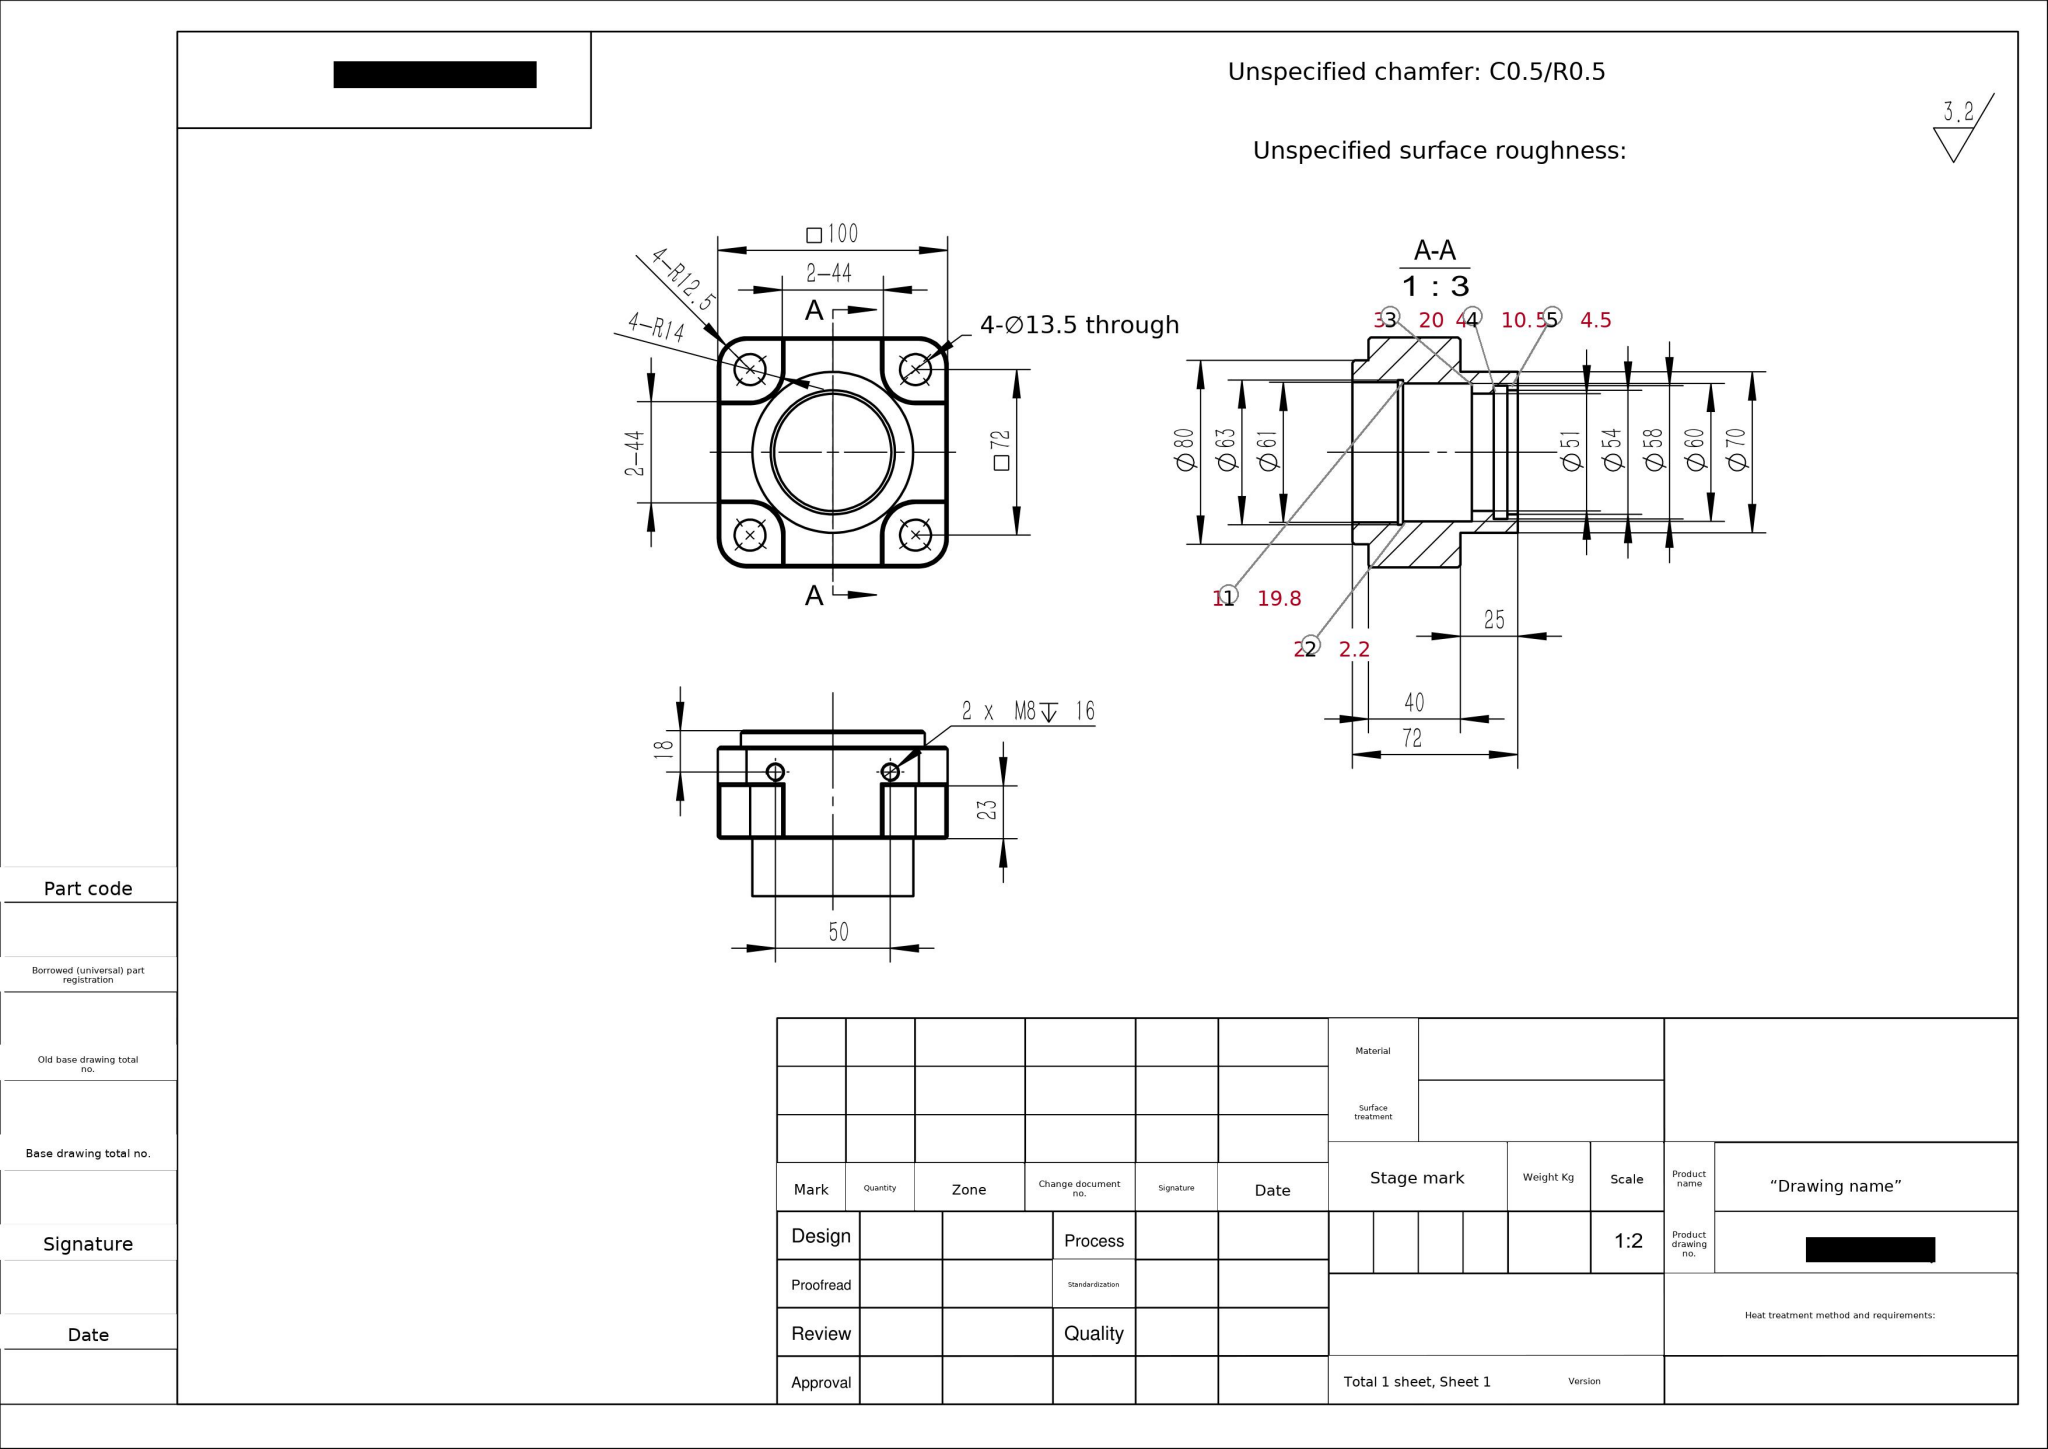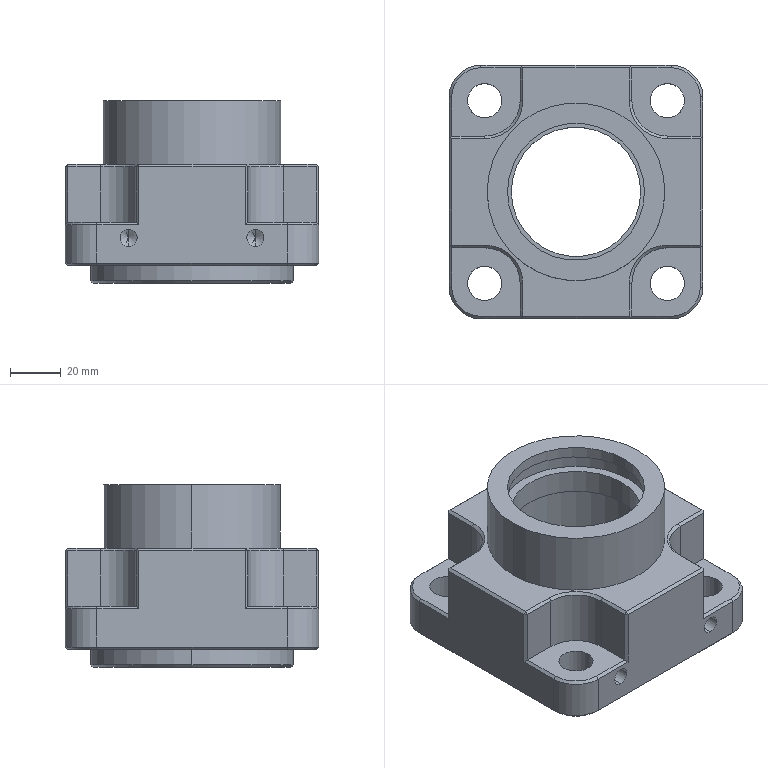Part | SolidWorks | mm | 1 solid | 113 faces | box 100 x 100 x 72 mm | volume 253658 mm3 | plane 59 | cylinder 36 | cone 18 | commonest cylinder face diameters 13.5 x8 6.8 x4 25 x4 28 x4 63 x2 61 x2 54 x2 58 x2